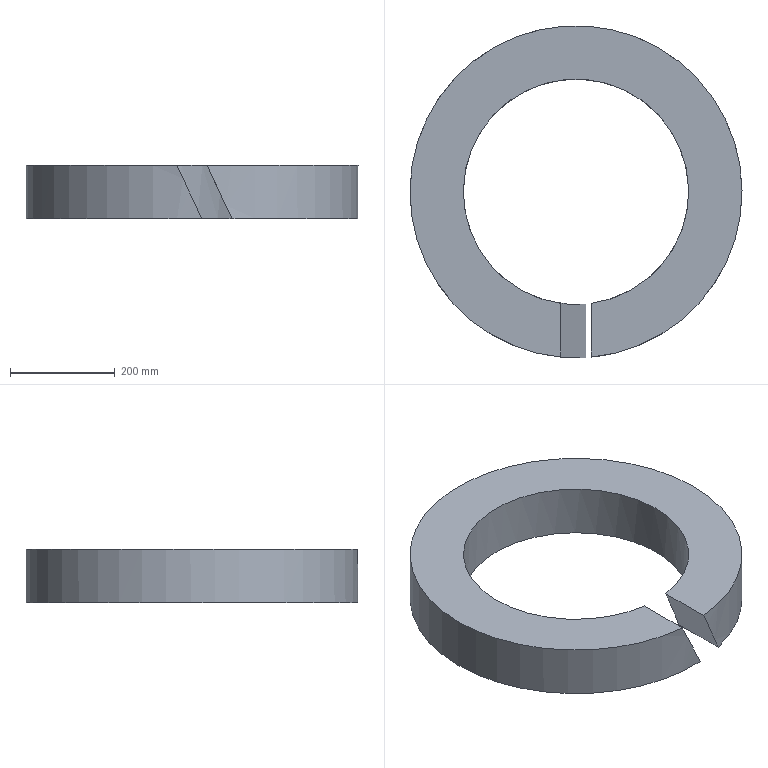Component | NX | 12 | 1 solid | 6 faces | volume 16617749 mm3 | plane 4 | cylinder 2 | commonest cylinder face diameters 429.26 x1 632.46 x1